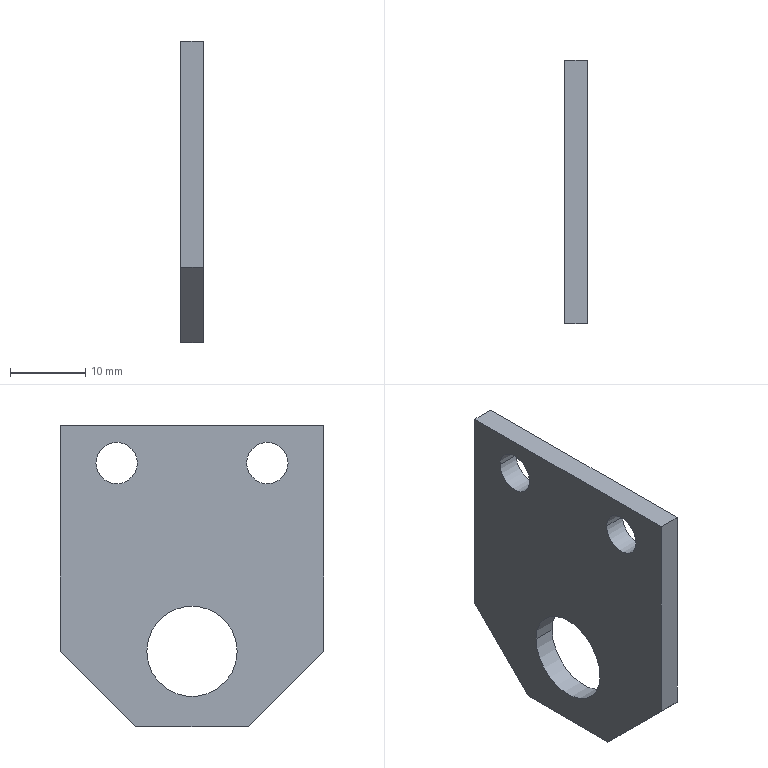Component | SolidWorks | ElectricalBoxAssembly2-1_AngleSensorComponentAssembly3-1_AngleDisplacementSensorMountingPlate-1 | 1 solid | 14 faces | box 3 x 35 x 40 mm | volume 3418 mm3 | plane 8 | cylinder 6 | commonest cylinder face diameters 5.5 x4 12 x2
build123d program:
from build123d import *

# Parameters (mm, degrees)
SKETCH1_W           = 35
SKETCH1_H           = 40
BOSS_EXTRUDE1_DEPTH = 3
SKETCH2_R           = 2.75
CUT_EXTRUDE1_DEPTH  = 27.744
SKETCH3_R           = 6
CUT_EXTRUDE2_DEPTH  = 27.744
CHAMFER1_SIZE       = 10


with BuildPart() as part:
    # Sketch1 → Boss-Extrude1 (new body)
    with BuildSketch(Plane.XY):
        Rectangle(SKETCH1_W, SKETCH1_H)
    extrude(amount=BOSS_EXTRUDE1_DEPTH)

    # Sketch2 → Cut-Extrude1 (cut, through all)
    with BuildSketch(Plane.XY.offset(3)):
        with Locations((-10, -15)):
            Circle(SKETCH2_R)
        with Locations((10, -15)):
            Circle(SKETCH2_R)
    extrude(amount=-CUT_EXTRUDE1_DEPTH, mode=Mode.SUBTRACT)

    # Sketch3 → Cut-Extrude2 (cut, through all)
    with BuildSketch(Plane.XY.offset(3)):
        with Locations((0, 10)):
            Circle(SKETCH3_R)
    extrude(amount=-CUT_EXTRUDE2_DEPTH, mode=Mode.SUBTRACT)

    # Chamfer1
    chamfer1_edges = [part.edges().sort_by_distance(p)[0] for p in [
        (-17.5, 20, 1.5),
        (17.5, 20, 1.5),
    ]]
    chamfer(chamfer1_edges, length=CHAMFER1_SIZE)


solid = part.part

# Placed as in the assembly
solid = solid.moved(Location((859.115, 214.666, 1756.399), (-90, 90, 0)))
STEP:
#1=COLOUR_RGB('',0.7922,0.8196,0.9333);
#2=FILL_AREA_STYLE_COLOUR('',#1);
#3=FILL_AREA_STYLE('',(#2));
#4=SURFACE_STYLE_FILL_AREA(#3);
#5=SURFACE_SIDE_STYLE('',(#4));
#6=SURFACE_STYLE_USAGE(.BOTH.,#5);
#7=PRESENTATION_STYLE_ASSIGNMENT((#6));
#8=CARTESIAN_POINT('',(33.942,8.215,68.756));
#9=VERTEX_POINT('',#8);
#10=CARTESIAN_POINT('',(33.942,8.688,68.756));
#11=VERTEX_POINT('',#10);
#12=CARTESIAN_POINT('',(33.942,8.451,68.756));
#13=DIRECTION('',(-1.,0.,0.));
#14=DIRECTION('',(0.,1.,0.));
#15=AXIS2_PLACEMENT_3D('',#12,#13,#14);
#16=CIRCLE('',#15,0.2362);
#17=EDGE_CURVE('',#9,#11,#16,.T.);
#18=ORIENTED_EDGE('',*,*,#17,.F.);
#19=CARTESIAN_POINT('',(33.823,8.215,68.756));
#20=VERTEX_POINT('',#19);
#21=CARTESIAN_POINT('',(33.942,8.215,68.756));
#22=DIRECTION('',(-1.,0.,0.));
#23=VECTOR('',#22,39.37);
#24=LINE('',#21,#23);
#25=EDGE_CURVE('',#9,#20,#24,.T.);
#26=ORIENTED_EDGE('',*,*,#25,.T.);
#27=CARTESIAN_POINT('',(33.823,8.688,68.756));
#28=VERTEX_POINT('',#27);
#29=CARTESIAN_POINT('',(33.823,8.451,68.756));
#30=DIRECTION('',(-1.,0.,0.));
#31=DIRECTION('',(0.,1.,0.));
#32=AXIS2_PLACEMENT_3D('',#29,#30,#31);
#33=CIRCLE('',#32,0.2362);
#34=EDGE_CURVE('',#20,#28,#33,.T.);
#35=ORIENTED_EDGE('',*,*,#34,.T.);
#36=CARTESIAN_POINT('',(33.942,8.688,68.756));
#37=DIRECTION('',(-1.,0.,0.));
#38=VECTOR('',#37,39.37);
#39=LINE('',#36,#38);
#40=EDGE_CURVE('',#11,#28,#39,.T.);
#41=ORIENTED_EDGE('',*,*,#40,.F.);
#42=EDGE_LOOP('',(#18,#26,#35,#41));
#43=FACE_OUTER_BOUND('',#42,.T.);
#44=CARTESIAN_POINT('',(33.942,8.451,68.756));
#45=DIRECTION('',(-1.,0.,0.));
#46=DIRECTION('',(0.,1.,0.));
#47=AXIS2_PLACEMENT_3D('',#44,#45,#46);
#48=CYLINDRICAL_SURFACE('',#47,0.2362);
#49=ADVANCED_FACE('',(#43),#48,.F.);
#50=CARTESIAN_POINT('',(33.942,8.737,69.74));
#51=VERTEX_POINT('',#50);
#52=CARTESIAN_POINT('',(33.942,8.953,69.74));
#53=VERTEX_POINT('',#52);
#54=CARTESIAN_POINT('',(33.942,8.845,69.74));
#55=DIRECTION('',(-1.,0.,0.));
#56=DIRECTION('',(0.,1.,0.));
#57=AXIS2_PLACEMENT_3D('',#54,#55,#56);
#58=CIRCLE('',#57,0.1083);
#59=EDGE_CURVE('',#51,#53,#58,.T.);
#60=ORIENTED_EDGE('',*,*,#59,.F.);
#61=CARTESIAN_POINT('',(33.823,8.737,69.74));
#62=VERTEX_POINT('',#61);
#63=CARTESIAN_POINT('',(33.942,8.737,69.74));
#64=DIRECTION('',(-1.,0.,0.));
#65=VECTOR('',#64,39.37);
#66=LINE('',#63,#65);
#67=EDGE_CURVE('',#51,#62,#66,.T.);
#68=ORIENTED_EDGE('',*,*,#67,.T.);
#69=CARTESIAN_POINT('',(33.823,8.953,69.74));
#70=VERTEX_POINT('',#69);
#71=CARTESIAN_POINT('',(33.823,8.845,69.74));
#72=DIRECTION('',(-1.,0.,0.));
#73=DIRECTION('',(0.,1.,0.));
#74=AXIS2_PLACEMENT_3D('',#71,#72,#73);
#75=CIRCLE('',#74,0.1083);
#76=EDGE_CURVE('',#62,#70,#75,.T.);
#77=ORIENTED_EDGE('',*,*,#76,.T.);
#78=CARTESIAN_POINT('',(33.942,8.953,69.74));
#79=DIRECTION('',(-1.,0.,0.));
#80=VECTOR('',#79,39.37);
#81=LINE('',#78,#80);
#82=EDGE_CURVE('',#53,#70,#81,.T.);
#83=ORIENTED_EDGE('',*,*,#82,.F.);
#84=EDGE_LOOP('',(#60,#68,#77,#83));
#85=FACE_OUTER_BOUND('',#84,.T.);
#86=CARTESIAN_POINT('',(33.942,8.845,69.74));
#87=DIRECTION('',(-1.,0.,0.));
#88=DIRECTION('',(0.,1.,0.));
#89=AXIS2_PLACEMENT_3D('',#86,#87,#88);
#90=CYLINDRICAL_SURFACE('',#89,0.1083);
#91=ADVANCED_FACE('',(#85),#90,.F.);
#92=CARTESIAN_POINT('',(33.942,7.949,69.74));
#93=VERTEX_POINT('',#92);
#94=CARTESIAN_POINT('',(33.942,8.166,69.74));
#95=VERTEX_POINT('',#94);
#96=CARTESIAN_POINT('',(33.942,8.058,69.74));
#97=DIRECTION('',(-1.,0.,0.));
#98=DIRECTION('',(0.,1.,0.));
#99=AXIS2_PLACEMENT_3D('',#96,#97,#98);
#100=CIRCLE('',#99,0.1083);
#101=EDGE_CURVE('',#93,#95,#100,.T.);
#102=ORIENTED_EDGE('',*,*,#101,.F.);
#103=CARTESIAN_POINT('',(33.823,7.949,69.74));
#104=VERTEX_POINT('',#103);
#105=CARTESIAN_POINT('',(33.942,7.949,69.74));
#106=DIRECTION('',(-1.,0.,0.));
#107=VECTOR('',#106,39.37);
#108=LINE('',#105,#107);
#109=EDGE_CURVE('',#93,#104,#108,.T.);
#110=ORIENTED_EDGE('',*,*,#109,.T.);
#111=CARTESIAN_POINT('',(33.823,8.166,69.74));
#112=VERTEX_POINT('',#111);
#113=CARTESIAN_POINT('',(33.823,8.058,69.74));
#114=DIRECTION('',(-1.,0.,0.));
#115=DIRECTION('',(0.,1.,0.));
#116=AXIS2_PLACEMENT_3D('',#113,#114,#115);
#117=CIRCLE('',#116,0.1083);
#118=EDGE_CURVE('',#104,#112,#117,.T.);
#119=ORIENTED_EDGE('',*,*,#118,.T.);
#120=CARTESIAN_POINT('',(33.942,8.166,69.74));
#121=DIRECTION('',(-1.,0.,0.));
#122=VECTOR('',#121,39.37);
#123=LINE('',#120,#122);
#124=EDGE_CURVE('',#95,#112,#123,.T.);
#125=ORIENTED_EDGE('',*,*,#124,.F.);
#126=EDGE_LOOP('',(#102,#110,#119,#125));
#127=FACE_OUTER_BOUND('',#126,.T.);
#128=CARTESIAN_POINT('',(33.942,8.058,69.74));
#129=DIRECTION('',(-1.,0.,0.));
#130=DIRECTION('',(0.,1.,0.));
#131=AXIS2_PLACEMENT_3D('',#128,#129,#130);
#132=CYLINDRICAL_SURFACE('',#131,0.1083);
#133=ADVANCED_FACE('',(#127),#132,.F.);
#134=CARTESIAN_POINT('',(33.942,9.14,69.937));
#135=VERTEX_POINT('',#134);
#136=CARTESIAN_POINT('',(33.942,9.14,68.756));
#137=VERTEX_POINT('',#136);
#138=CARTESIAN_POINT('',(33.942,9.14,68.362));
#139=DIRECTION('',(-0.,-0.,-1.));
#140=VECTOR('',#139,39.37);
#141=LINE('',#138,#140);
#142=EDGE_CURVE('',#135,#137,#141,.T.);
#143=ORIENTED_EDGE('',*,*,#142,.T.);
#144=CARTESIAN_POINT('',(33.823,9.14,68.756));
#145=VERTEX_POINT('',#144);
#146=CARTESIAN_POINT('',(33.823,9.14,68.756));
#147=DIRECTION('',(-1.,0.,0.));
#148=VECTOR('',#147,39.37);
#149=LINE('',#146,#148);
#150=EDGE_CURVE('',#137,#145,#149,.T.);
#151=ORIENTED_EDGE('',*,*,#150,.T.);
#152=CARTESIAN_POINT('',(33.823,9.14,69.937));
#153=VERTEX_POINT('',#152);
#154=CARTESIAN_POINT('',(33.823,9.14,68.362));
#155=DIRECTION('',(-0.,-0.,-1.));
#156=VECTOR('',#155,39.37);
#157=LINE('',#154,#156);
#158=EDGE_CURVE('',#153,#145,#157,.T.);
#159=ORIENTED_EDGE('',*,*,#158,.F.);
#160=CARTESIAN_POINT('',(33.823,9.14,69.937));
#161=DIRECTION('',(1.,-0.,-0.));
#162=VECTOR('',#161,39.37);
#163=LINE('',#160,#162);
#164=EDGE_CURVE('',#153,#135,#163,.T.);
#165=ORIENTED_EDGE('',*,*,#164,.T.);
#166=EDGE_LOOP('',(#143,#151,#159,#165));
#167=FACE_OUTER_BOUND('',#166,.T.);
#168=CARTESIAN_POINT('',(33.823,9.14,68.362));
#169=DIRECTION('',(-0.,-1.,0.));
#170=DIRECTION('',(0.,0.,1.));
#171=AXIS2_PLACEMENT_3D('',#168,#169,#170);
#172=PLANE('',#171);
#173=ADVANCED_FACE('',(#167),#172,.F.);
#174=CARTESIAN_POINT('',(33.823,8.747,68.362));
#175=VERTEX_POINT('',#174);
#176=CARTESIAN_POINT('',(33.823,8.156,68.362));
#177=VERTEX_POINT('',#176);
#178=CARTESIAN_POINT('',(33.823,7.762,68.362));
#179=DIRECTION('',(-0.,-1.,0.));
#180=VECTOR('',#179,39.37);
#181=LINE('',#178,#180);
#182=EDGE_CURVE('',#175,#177,#181,.T.);
#183=ORIENTED_EDGE('',*,*,#182,.F.);
#184=CARTESIAN_POINT('',(33.942,8.747,68.362));
#185=VERTEX_POINT('',#184);
#186=CARTESIAN_POINT('',(33.823,8.747,68.362));
#187=DIRECTION('',(1.,-0.,-0.));
#188=VECTOR('',#187,39.37);
#189=LINE('',#186,#188);
#190=EDGE_CURVE('',#175,#185,#189,.T.);
#191=ORIENTED_EDGE('',*,*,#190,.T.);
#192=CARTESIAN_POINT('',(33.942,8.156,68.362));
#193=VERTEX_POINT('',#192);
#194=CARTESIAN_POINT('',(33.942,7.762,68.362));
#195=DIRECTION('',(-0.,-1.,0.));
#196=VECTOR('',#195,39.37);
#197=LINE('',#194,#196);
#198=EDGE_CURVE('',#185,#193,#197,.T.);
#199=ORIENTED_EDGE('',*,*,#198,.T.);
#200=CARTESIAN_POINT('',(33.823,8.156,68.362));
#201=DIRECTION('',(-1.,0.,0.));
#202=VECTOR('',#201,39.37);
#203=LINE('',#200,#202);
#204=EDGE_CURVE('',#193,#177,#203,.T.);
#205=ORIENTED_EDGE('',*,*,#204,.T.);
#206=EDGE_LOOP('',(#183,#191,#199,#205));
#207=FACE_OUTER_BOUND('',#206,.T.);
#208=CARTESIAN_POINT('',(33.823,7.762,68.362));
#209=DIRECTION('',(0.,0.,1.));
#210=DIRECTION('',(1.,-0.,-0.));
#211=AXIS2_PLACEMENT_3D('',#208,#209,#210);
#212=PLANE('',#211);
#213=ADVANCED_FACE('',(#207),#212,.F.);
#214=CARTESIAN_POINT('',(33.823,7.762,68.756));
#215=VERTEX_POINT('',#214);
#216=CARTESIAN_POINT('',(33.823,7.762,69.937));
#217=VERTEX_POINT('',#216);
#218=CARTESIAN_POINT('',(33.823,7.762,68.362));
#219=DIRECTION('',(0.,0.,1.));
#220=VECTOR('',#219,39.37);
#221=LINE('',#218,#220);
#222=EDGE_CURVE('',#215,#217,#221,.T.);
#223=ORIENTED_EDGE('',*,*,#222,.F.);
#224=CARTESIAN_POINT('',(33.942,7.762,68.756));
#225=VERTEX_POINT('',#224);
#226=CARTESIAN_POINT('',(33.823,7.762,68.756));
#227=DIRECTION('',(1.,-0.,-0.));
#228=VECTOR('',#227,39.37);
#229=LINE('',#226,#228);
#230=EDGE_CURVE('',#215,#225,#229,.T.);
#231=ORIENTED_EDGE('',*,*,#230,.T.);
#232=CARTESIAN_POINT('',(33.942,7.762,69.937));
#233=VERTEX_POINT('',#232);
#234=CARTESIAN_POINT('',(33.942,7.762,68.362));
#235=DIRECTION('',(0.,0.,1.));
#236=VECTOR('',#235,39.37);
#237=LINE('',#234,#236);
#238=EDGE_CURVE('',#225,#233,#237,.T.);
#239=ORIENTED_EDGE('',*,*,#238,.T.);
#240=CARTESIAN_POINT('',(33.823,7.762,69.937));
#241=DIRECTION('',(1.,-0.,-0.));
#242=VECTOR('',#241,39.37);
#243=LINE('',#240,#242);
#244=EDGE_CURVE('',#217,#233,#243,.T.);
#245=ORIENTED_EDGE('',*,*,#244,.F.);
#246=EDGE_LOOP('',(#223,#231,#239,#245));
#247=FACE_OUTER_BOUND('',#246,.T.);
#248=CARTESIAN_POINT('',(33.823,7.762,68.362));
#249=DIRECTION('',(0.,1.,-0.));
#250=DIRECTION('',(-0.,-0.,-1.));
#251=AXIS2_PLACEMENT_3D('',#248,#249,#250);
#252=PLANE('',#251);
#253=ADVANCED_FACE('',(#247),#252,.F.);
#254=CARTESIAN_POINT('',(33.942,7.762,69.937));
#255=DIRECTION('',(0.,1.,-0.));
#256=VECTOR('',#255,39.37);
#257=LINE('',#254,#256);
#258=EDGE_CURVE('',#233,#135,#257,.T.);
#259=ORIENTED_EDGE('',*,*,#258,.T.);
#260=ORIENTED_EDGE('',*,*,#164,.F.);
#261=CARTESIAN_POINT('',(33.823,7.762,69.937));
#262=DIRECTION('',(0.,1.,-0.));
#263=VECTOR('',#262,39.37);
#264=LINE('',#261,#263);
#265=EDGE_CURVE('',#217,#153,#264,.T.);
#266=ORIENTED_EDGE('',*,*,#265,.F.);
#267=ORIENTED_EDGE('',*,*,#244,.T.);
#268=EDGE_LOOP('',(#259,#260,#266,#267));
#269=FACE_OUTER_BOUND('',#268,.T.);
#270=CARTESIAN_POINT('',(33.823,7.762,69.937));
#271=DIRECTION('',(-0.,-0.,-1.));
#272=DIRECTION('',(-1.,0.,0.));
#273=AXIS2_PLACEMENT_3D('',#270,#271,#272);
#274=PLANE('',#273);
#275=ADVANCED_FACE('',(#269),#274,.F.);
#276=CARTESIAN_POINT('',(33.823,8.451,68.756));
#277=DIRECTION('',(-1.,0.,0.));
#278=DIRECTION('',(0.,1.,0.));
#279=AXIS2_PLACEMENT_3D('',#276,#277,#278);
#280=CIRCLE('',#279,0.2362);
#281=EDGE_CURVE('',#28,#20,#280,.T.);
#282=ORIENTED_EDGE('',*,*,#281,.F.);
#283=ORIENTED_EDGE('',*,*,#34,.F.);
#284=EDGE_LOOP('',(#282,#283));
#285=FACE_BOUND('',#284,.T.);
#286=CARTESIAN_POINT('',(33.823,8.845,69.74));
#287=DIRECTION('',(-1.,0.,0.));
#288=DIRECTION('',(0.,1.,0.));
#289=AXIS2_PLACEMENT_3D('',#286,#287,#288);
#290=CIRCLE('',#289,0.1083);
#291=EDGE_CURVE('',#70,#62,#290,.T.);
#292=ORIENTED_EDGE('',*,*,#291,.F.);
#293=ORIENTED_EDGE('',*,*,#76,.F.);
#294=EDGE_LOOP('',(#292,#293));
#295=FACE_BOUND('',#294,.T.);
#296=CARTESIAN_POINT('',(33.823,8.058,69.74));
#297=DIRECTION('',(-1.,0.,0.));
#298=DIRECTION('',(0.,1.,0.));
#299=AXIS2_PLACEMENT_3D('',#296,#297,#298);
#300=CIRCLE('',#299,0.1083);
#301=EDGE_CURVE('',#112,#104,#300,.T.);
#302=ORIENTED_EDGE('',*,*,#301,.F.);
#303=ORIENTED_EDGE('',*,*,#118,.F.);
#304=EDGE_LOOP('',(#302,#303));
#305=FACE_BOUND('',#304,.T.);
#306=ORIENTED_EDGE('',*,*,#158,.T.);
#307=CARTESIAN_POINT('',(33.823,8.993,68.608));
#308=DIRECTION('',(-0.,-0.7071,-0.7071));
#309=VECTOR('',#308,39.37);
#310=LINE('',#307,#309);
#311=EDGE_CURVE('',#145,#175,#310,.T.);
#312=ORIENTED_EDGE('',*,*,#311,.T.);
#313=ORIENTED_EDGE('',*,*,#182,.T.);
#314=CARTESIAN_POINT('',(33.823,7.91,68.608));
#315=DIRECTION('',(0.,-0.7071,0.7071));
#316=VECTOR('',#315,39.37);
#317=LINE('',#314,#316);
#318=EDGE_CURVE('',#177,#215,#317,.T.);
#319=ORIENTED_EDGE('',*,*,#318,.T.);
#320=ORIENTED_EDGE('',*,*,#222,.T.);
#321=ORIENTED_EDGE('',*,*,#265,.T.);
#322=EDGE_LOOP('',(#306,#312,#313,#319,#320,#321));
#323=FACE_OUTER_BOUND('',#322,.T.);
#324=CARTESIAN_POINT('',(33.823,8.451,69.15));
#325=DIRECTION('',(-1.,0.,0.));
#326=DIRECTION('',(0.,1.,-0.));
#327=AXIS2_PLACEMENT_3D('',#324,#325,#326);
#328=PLANE('',#327);
#329=ADVANCED_FACE('',(#285,#295,#305,#323),#328,.T.);
#330=CARTESIAN_POINT('',(33.942,8.451,68.756));
#331=DIRECTION('',(-1.,0.,0.));
#332=DIRECTION('',(0.,1.,0.));
#333=AXIS2_PLACEMENT_3D('',#330,#331,#332);
#334=CIRCLE('',#333,0.2362);
#335=EDGE_CURVE('',#11,#9,#334,.T.);
#336=ORIENTED_EDGE('',*,*,#335,.T.);
#337=ORIENTED_EDGE('',*,*,#17,.T.);
#338=EDGE_LOOP('',(#336,#337));
#339=FACE_BOUND('',#338,.T.);
#340=CARTESIAN_POINT('',(33.942,8.845,69.74));
#341=DIRECTION('',(-1.,0.,0.));
#342=DIRECTION('',(0.,1.,0.));
#343=AXIS2_PLACEMENT_3D('',#340,#341,#342);
#344=CIRCLE('',#343,0.1083);
#345=EDGE_CURVE('',#53,#51,#344,.T.);
#346=ORIENTED_EDGE('',*,*,#345,.T.);
#347=ORIENTED_EDGE('',*,*,#59,.T.);
#348=EDGE_LOOP('',(#346,#347));
#349=FACE_BOUND('',#348,.T.);
#350=CARTESIAN_POINT('',(33.942,8.058,69.74));
#351=DIRECTION('',(-1.,0.,0.));
#352=DIRECTION('',(0.,1.,0.));
#353=AXIS2_PLACEMENT_3D('',#350,#351,#352);
#354=CIRCLE('',#353,0.1083);
#355=EDGE_CURVE('',#95,#93,#354,.T.);
#356=ORIENTED_EDGE('',*,*,#355,.T.);
#357=ORIENTED_EDGE('',*,*,#101,.T.);
#358=EDGE_LOOP('',(#356,#357));
#359=FACE_BOUND('',#358,.T.);
#360=ORIENTED_EDGE('',*,*,#198,.F.);
#361=CARTESIAN_POINT('',(33.942,8.747,68.362));
#362=DIRECTION('',(0.,0.7071,0.7071));
#363=VECTOR('',#362,39.37);
#364=LINE('',#361,#363);
#365=EDGE_CURVE('',#185,#137,#364,.T.);
#366=ORIENTED_EDGE('',*,*,#365,.T.);
#367=ORIENTED_EDGE('',*,*,#142,.F.);
#368=ORIENTED_EDGE('',*,*,#258,.F.);
#369=ORIENTED_EDGE('',*,*,#238,.F.);
#370=CARTESIAN_POINT('',(33.942,7.762,68.756));
#371=DIRECTION('',(-0.,0.7071,-0.7071));
#372=VECTOR('',#371,39.37);
#373=LINE('',#370,#372);
#374=EDGE_CURVE('',#225,#193,#373,.T.);
#375=ORIENTED_EDGE('',*,*,#374,.T.);
#376=EDGE_LOOP('',(#360,#366,#367,#368,#369,#375));
#377=FACE_OUTER_BOUND('',#376,.T.);
#378=CARTESIAN_POINT('',(33.942,8.451,69.15));
#379=DIRECTION('',(-1.,0.,0.));
#380=DIRECTION('',(0.,1.,-0.));
#381=AXIS2_PLACEMENT_3D('',#378,#379,#380);
#382=PLANE('',#381);
#383=ADVANCED_FACE('',(#339,#349,#359,#377),#382,.F.);
#384=ORIENTED_EDGE('',*,*,#109,.F.);
#385=ORIENTED_EDGE('',*,*,#355,.F.);
#386=ORIENTED_EDGE('',*,*,#124,.T.);
#387=ORIENTED_EDGE('',*,*,#301,.T.);
#388=EDGE_LOOP('',(#384,#385,#386,#387));
#389=FACE_OUTER_BOUND('',#388,.T.);
#390=CARTESIAN_POINT('',(33.942,8.058,69.74));
#391=DIRECTION('',(-1.,0.,0.));
#392=DIRECTION('',(0.,1.,0.));
#393=AXIS2_PLACEMENT_3D('',#390,#391,#392);
#394=CYLINDRICAL_SURFACE('',#393,0.1083);
#395=ADVANCED_FACE('',(#389),#394,.F.);
#396=ORIENTED_EDGE('',*,*,#67,.F.);
#397=ORIENTED_EDGE('',*,*,#345,.F.);
#398=ORIENTED_EDGE('',*,*,#82,.T.);
#399=ORIENTED_EDGE('',*,*,#291,.T.);
#400=EDGE_LOOP('',(#396,#397,#398,#399));
#401=FACE_OUTER_BOUND('',#400,.T.);
#402=CARTESIAN_POINT('',(33.942,8.845,69.74));
#403=DIRECTION('',(-1.,0.,0.));
#404=DIRECTION('',(0.,1.,0.));
#405=AXIS2_PLACEMENT_3D('',#402,#403,#404);
#406=CYLINDRICAL_SURFACE('',#405,0.1083);
#407=ADVANCED_FACE('',(#401),#406,.F.);
#408=ORIENTED_EDGE('',*,*,#25,.F.);
#409=ORIENTED_EDGE('',*,*,#335,.F.);
#410=ORIENTED_EDGE('',*,*,#40,.T.);
#411=ORIENTED_EDGE('',*,*,#281,.T.);
#412=EDGE_LOOP('',(#408,#409,#410,#411));
#413=FACE_OUTER_BOUND('',#412,.T.);
#414=CARTESIAN_POINT('',(33.942,8.451,68.756));
#415=DIRECTION('',(-1.,0.,0.));
#416=DIRECTION('',(0.,1.,0.));
#417=AXIS2_PLACEMENT_3D('',#414,#415,#416);
#418=CYLINDRICAL_SURFACE('',#417,0.2362);
#419=ADVANCED_FACE('',(#413),#418,.F.);
#420=ORIENTED_EDGE('',*,*,#311,.F.);
#421=ORIENTED_EDGE('',*,*,#150,.F.);
#422=ORIENTED_EDGE('',*,*,#365,.F.);
#423=ORIENTED_EDGE('',*,*,#190,.F.);
#424=EDGE_LOOP('',(#420,#421,#422,#423));
#425=FACE_OUTER_BOUND('',#424,.T.);
#426=CARTESIAN_POINT('',(33.823,8.747,68.362));
#427=DIRECTION('',(0.,-0.7071,0.7071));
#428=DIRECTION('',(1.,-0.,-0.));
#429=AXIS2_PLACEMENT_3D('',#426,#427,#428);
#430=PLANE('',#429);
#431=ADVANCED_FACE('',(#425),#430,.F.);
#432=ORIENTED_EDGE('',*,*,#318,.F.);
#433=ORIENTED_EDGE('',*,*,#204,.F.);
#434=ORIENTED_EDGE('',*,*,#374,.F.);
#435=ORIENTED_EDGE('',*,*,#230,.F.);
#436=EDGE_LOOP('',(#432,#433,#434,#435));
#437=FACE_OUTER_BOUND('',#436,.T.);
#438=CARTESIAN_POINT('',(33.823,7.762,68.756));
#439=DIRECTION('',(0.,0.7071,0.7071));
#440=DIRECTION('',(1.,-0.,-0.));
#441=AXIS2_PLACEMENT_3D('',#438,#439,#440);
#442=PLANE('',#441);
#443=ADVANCED_FACE('',(#437),#442,.F.);
#444=CLOSED_SHELL('',(#49,#91,#133,#173,#213,#253,#275,#329,#383,#395,#407,#419,#431,#443));
#445=MANIFOLD_SOLID_BREP('',#444);
#446=STYLED_ITEM('',(#7),#445);
#447=(LENGTH_UNIT()NAMED_UNIT(*)SI_UNIT($,.METRE.));
#448=LENGTH_MEASURE_WITH_UNIT(LENGTH_MEASURE(0.0254),#447);
#449=DIMENSIONAL_EXPONENTS(1.,0.,0.,0.,0.,0.,0.);
#450=(CONVERSION_BASED_UNIT('',#448)LENGTH_UNIT()NAMED_UNIT(#449));
#451=UNCERTAINTY_MEASURE_WITH_UNIT(LENGTH_MEASURE(0.00001),#450,'','');
#452=(NAMED_UNIT(*)PLANE_ANGLE_UNIT()SI_UNIT($,.RADIAN.));
#453=(NAMED_UNIT(*)SI_UNIT($,.STERADIAN.)SOLID_ANGLE_UNIT());
#454=(GEOMETRIC_REPRESENTATION_CONTEXT(3)GLOBAL_UNCERTAINTY_ASSIGNED_CONTEXT((#451))GLOBAL_UNIT_ASSIGNED_CONTEXT((#450,#452,#453))REPRESENTATION_CONTEXT('',''));
#455=MECHANICAL_DESIGN_GEOMETRIC_PRESENTATION_REPRESENTATION('',(#446),#454);
#456=CARTESIAN_POINT('',(0.,0.,0.));
#457=DIRECTION('',(0.,0.,1.));
#458=DIRECTION('',(1.,0.,0.));
#459=AXIS2_PLACEMENT_3D('',#456,#457,#458);
#460=(LENGTH_UNIT()NAMED_UNIT(*)SI_UNIT($,.METRE.));
#461=LENGTH_MEASURE_WITH_UNIT(LENGTH_MEASURE(0.0254),#460);
#462=DIMENSIONAL_EXPONENTS(1.,0.,0.,0.,0.,0.,0.);
#463=(CONVERSION_BASED_UNIT('',#461)LENGTH_UNIT()NAMED_UNIT(#462));
#464=UNCERTAINTY_MEASURE_WITH_UNIT(LENGTH_MEASURE(0.00001),#463,'','');
#465=(NAMED_UNIT(*)PLANE_ANGLE_UNIT()SI_UNIT($,.RADIAN.));
#466=(NAMED_UNIT(*)SI_UNIT($,.STERADIAN.)SOLID_ANGLE_UNIT());
#467=(GEOMETRIC_REPRESENTATION_CONTEXT(3)GLOBAL_UNCERTAINTY_ASSIGNED_CONTEXT((#464))GLOBAL_UNIT_ASSIGNED_CONTEXT((#463,#465,#466))REPRESENTATION_CONTEXT('',''));
#468=ADVANCED_BREP_SHAPE_REPRESENTATION('',(#445,#459),#467);
#469=PRESENTATION_LAYER_ASSIGNMENT('','',(#446));